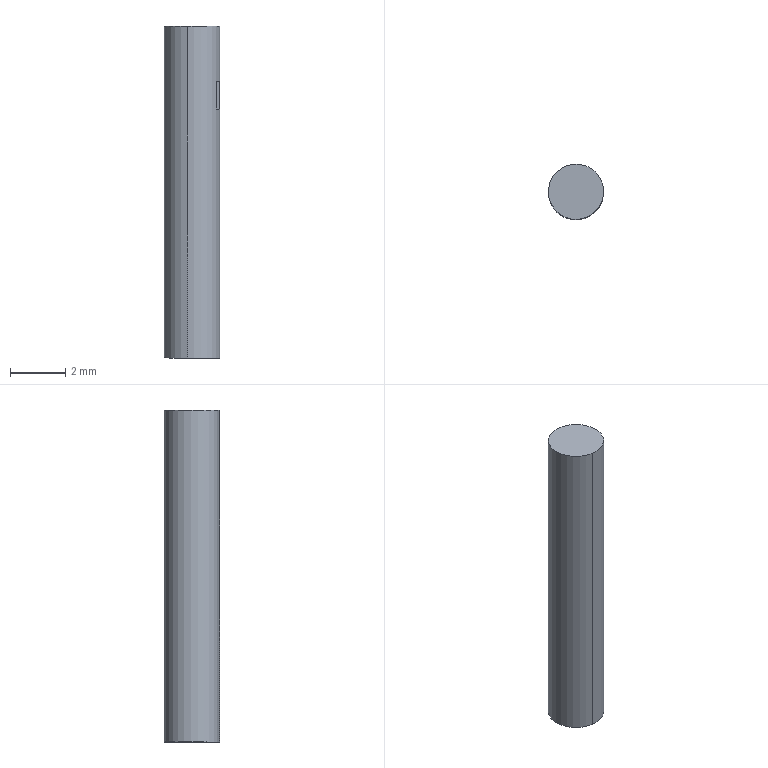Component | SolidWorks | RearAxis-1 | 1 solid | 9 faces | box 2 x 2 x 12 mm | volume 38 mm3 | plane 7 | cylinder 2 | commonest cylinder face diameters 2 x2
build123d program:
from build123d import *

# Parameters (mm, degrees)
BOSS_EXTRUDE1_DEPTH      = 5
BOSS_EXTRUDE1_DEPTH_BACK = 7
SKETCH2_R                = 1
CUT_EXTRUDE1_START       = -2
SKETCH3_W                = 0.7
SKETCH3_H                = 0.5
CUT_EXTRUDE1_DEPTH       = 1


with BuildPart() as part:
    # Sketch2 → Boss-Extrude1 (new, two sides: drawn at the far end of the back side and taken through both)
    with BuildSketch(Plane.XY.offset(-BOSS_EXTRUDE1_DEPTH_BACK)):
        with Locations((-5, 0)):
            Circle(SKETCH2_R)
    extrude(amount=BOSS_EXTRUDE1_DEPTH + BOSS_EXTRUDE1_DEPTH_BACK)

    # Sketch3 → Cut-Extrude1 (cut)
    with BuildSketch(Plane.XY.offset(5).offset(CUT_EXTRUDE1_START)):
        with Locations((-5, 1)):
            Rectangle(SKETCH3_W, SKETCH3_H)
    extrude(amount=-CUT_EXTRUDE1_DEPTH, mode=Mode.SUBTRACT)


solid = part.part

# Placed as in the assembly
solid = solid.moved(Location((11.697, -8.435, 2), (0, 0, -99.237)))
STEP:
#1=CARTESIAN_POINT('',(0.5307,-0.1301,0.1575));
#2=VERTEX_POINT('',#1);
#3=CARTESIAN_POINT('',(0.5307,-0.1301,0.1969));
#4=VERTEX_POINT('',#3);
#5=CARTESIAN_POINT('',(0.5307,-0.1301,-0.1969));
#6=DIRECTION('',(0.,-0.,1.));
#7=VECTOR('',#6,39.37);
#8=LINE('',#5,#7);
#9=EDGE_CURVE('',#2,#4,#8,.T.);
#10=ORIENTED_EDGE('',*,*,#9,.F.);
#11=CARTESIAN_POINT('',(0.5263,-0.1573,0.1575));
#12=VERTEX_POINT('',#11);
#13=CARTESIAN_POINT('',(0.4921,-0.1378,0.1575));
#14=DIRECTION('',(-0.,0.,-1.));
#15=DIRECTION('',(-0.1605,-0.987,0.));
#16=AXIS2_PLACEMENT_3D('',#13,#14,#15);
#17=CIRCLE('',#16,0.03937);
#18=EDGE_CURVE('',#2,#12,#17,.T.);
#19=ORIENTED_EDGE('',*,*,#18,.T.);
#20=CARTESIAN_POINT('',(0.5263,-0.1573,0.1969));
#21=VERTEX_POINT('',#20);
#22=CARTESIAN_POINT('',(0.5263,-0.1573,-0.1969));
#23=DIRECTION('',(-0.,0.,-1.));
#24=VECTOR('',#23,39.37);
#25=LINE('',#22,#24);
#26=EDGE_CURVE('',#21,#12,#25,.T.);
#27=ORIENTED_EDGE('',*,*,#26,.F.);
#28=CARTESIAN_POINT('',(0.4921,-0.1378,0.1969));
#29=DIRECTION('',(-0.,0.,-1.));
#30=DIRECTION('',(-0.1605,-0.987,0.));
#31=AXIS2_PLACEMENT_3D('',#28,#29,#30);
#32=CIRCLE('',#31,0.03937);
#33=EDGE_CURVE('',#4,#21,#32,.T.);
#34=ORIENTED_EDGE('',*,*,#33,.F.);
#35=EDGE_LOOP('',(#10,#19,#27,#34));
#36=FACE_BOUND('',#35,.T.);
#37=CARTESIAN_POINT('',(0.4858,-0.1767,-0.1969));
#38=VERTEX_POINT('',#37);
#39=CARTESIAN_POINT('',(0.4984,-0.09894,-0.1969));
#40=VERTEX_POINT('',#39);
#41=CARTESIAN_POINT('',(0.4921,-0.1378,-0.1969));
#42=DIRECTION('',(0.,-0.,1.));
#43=DIRECTION('',(-0.1605,-0.987,0.));
#44=AXIS2_PLACEMENT_3D('',#41,#42,#43);
#45=CIRCLE('',#44,0.03937);
#46=EDGE_CURVE('',#38,#40,#45,.T.);
#47=ORIENTED_EDGE('',*,*,#46,.T.);
#48=CARTESIAN_POINT('',(0.4984,-0.09894,0.2756));
#49=VERTEX_POINT('',#48);
#50=CARTESIAN_POINT('',(0.4984,-0.09894,-0.1969));
#51=DIRECTION('',(0.,-0.,1.));
#52=VECTOR('',#51,39.37);
#53=LINE('',#50,#52);
#54=EDGE_CURVE('',#40,#49,#53,.T.);
#55=ORIENTED_EDGE('',*,*,#54,.T.);
#56=CARTESIAN_POINT('',(0.4858,-0.1767,0.2756));
#57=VERTEX_POINT('',#56);
#58=CARTESIAN_POINT('',(0.4921,-0.1378,0.2756));
#59=DIRECTION('',(0.,-0.,1.));
#60=DIRECTION('',(-0.1605,-0.987,0.));
#61=AXIS2_PLACEMENT_3D('',#58,#59,#60);
#62=CIRCLE('',#61,0.03937);
#63=EDGE_CURVE('',#57,#49,#62,.T.);
#64=ORIENTED_EDGE('',*,*,#63,.F.);
#65=CARTESIAN_POINT('',(0.4858,-0.1767,-0.1969));
#66=DIRECTION('',(0.,-0.,1.));
#67=VECTOR('',#66,39.37);
#68=LINE('',#65,#67);
#69=EDGE_CURVE('',#38,#57,#68,.T.);
#70=ORIENTED_EDGE('',*,*,#69,.F.);
#71=EDGE_LOOP('',(#47,#55,#64,#70));
#72=FACE_OUTER_BOUND('',#71,.T.);
#73=CARTESIAN_POINT('',(0.4921,-0.1378,-0.1969));
#74=DIRECTION('',(0.,-0.,1.));
#75=DIRECTION('',(-0.1605,-0.987,0.));
#76=AXIS2_PLACEMENT_3D('',#73,#74,#75);
#77=CYLINDRICAL_SURFACE('',#76,0.03937);
#78=ADVANCED_FACE('',(#36,#72),#77,.T.);
#79=ORIENTED_EDGE('',*,*,#54,.F.);
#80=CARTESIAN_POINT('',(0.4921,-0.1378,-0.1969));
#81=DIRECTION('',(0.,-0.,1.));
#82=DIRECTION('',(-0.1605,-0.987,0.));
#83=AXIS2_PLACEMENT_3D('',#80,#81,#82);
#84=CIRCLE('',#83,0.03937);
#85=EDGE_CURVE('',#40,#38,#84,.T.);
#86=ORIENTED_EDGE('',*,*,#85,.T.);
#87=ORIENTED_EDGE('',*,*,#69,.T.);
#88=CARTESIAN_POINT('',(0.4921,-0.1378,0.2756));
#89=DIRECTION('',(0.,-0.,1.));
#90=DIRECTION('',(-0.1605,-0.987,0.));
#91=AXIS2_PLACEMENT_3D('',#88,#89,#90);
#92=CIRCLE('',#91,0.03937);
#93=EDGE_CURVE('',#49,#57,#92,.T.);
#94=ORIENTED_EDGE('',*,*,#93,.F.);
#95=EDGE_LOOP('',(#79,#86,#87,#94));
#96=FACE_OUTER_BOUND('',#95,.T.);
#97=CARTESIAN_POINT('',(0.4921,-0.1378,-0.1969));
#98=DIRECTION('',(0.,-0.,1.));
#99=DIRECTION('',(-0.1605,-0.987,0.));
#100=AXIS2_PLACEMENT_3D('',#97,#98,#99);
#101=CYLINDRICAL_SURFACE('',#100,0.03937);
#102=ADVANCED_FACE('',(#96),#101,.T.);
#103=ORIENTED_EDGE('',*,*,#46,.F.);
#104=ORIENTED_EDGE('',*,*,#85,.F.);
#105=EDGE_LOOP('',(#103,#104));
#106=FACE_OUTER_BOUND('',#105,.T.);
#107=CARTESIAN_POINT('',(0.4921,-0.1378,-0.1969));
#108=DIRECTION('',(0.,-0.,1.));
#109=DIRECTION('',(-0.1605,-0.987,-0.));
#110=AXIS2_PLACEMENT_3D('',#107,#108,#109);
#111=PLANE('',#110);
#112=ADVANCED_FACE('',(#106),#111,.F.);
#113=ORIENTED_EDGE('',*,*,#63,.T.);
#114=ORIENTED_EDGE('',*,*,#93,.T.);
#115=EDGE_LOOP('',(#113,#114));
#116=FACE_OUTER_BOUND('',#115,.T.);
#117=CARTESIAN_POINT('',(0.4921,-0.1378,0.2756));
#118=DIRECTION('',(0.,-0.,1.));
#119=DIRECTION('',(-0.1605,-0.987,-0.));
#120=AXIS2_PLACEMENT_3D('',#117,#118,#119);
#121=PLANE('',#120);
#122=ADVANCED_FACE('',(#116),#121,.T.);
#123=ORIENTED_EDGE('',*,*,#26,.T.);
#124=CARTESIAN_POINT('',(0.5191,-0.1561,0.1575));
#125=VERTEX_POINT('',#124);
#126=CARTESIAN_POINT('',(0.5385,-0.1593,0.1575));
#127=DIRECTION('',(0.987,-0.1605,-0.));
#128=VECTOR('',#127,39.37);
#129=LINE('',#126,#128);
#130=EDGE_CURVE('',#125,#12,#129,.T.);
#131=ORIENTED_EDGE('',*,*,#130,.F.);
#132=CARTESIAN_POINT('',(0.5191,-0.1561,0.1969));
#133=VERTEX_POINT('',#132);
#134=CARTESIAN_POINT('',(0.5191,-0.1561,0.1575));
#135=DIRECTION('',(0.,-0.,1.));
#136=VECTOR('',#135,39.37);
#137=LINE('',#134,#136);
#138=EDGE_CURVE('',#125,#133,#137,.T.);
#139=ORIENTED_EDGE('',*,*,#138,.T.);
#140=CARTESIAN_POINT('',(0.5385,-0.1593,0.1969));
#141=DIRECTION('',(0.987,-0.1605,-0.));
#142=VECTOR('',#141,39.37);
#143=LINE('',#140,#142);
#144=EDGE_CURVE('',#133,#21,#143,.T.);
#145=ORIENTED_EDGE('',*,*,#144,.T.);
#146=EDGE_LOOP('',(#123,#131,#139,#145));
#147=FACE_OUTER_BOUND('',#146,.T.);
#148=CARTESIAN_POINT('',(0.5385,-0.1593,0.1575));
#149=DIRECTION('',(-0.1605,-0.987,-0.));
#150=DIRECTION('',(-0.,0.,-1.));
#151=AXIS2_PLACEMENT_3D('',#148,#149,#150);
#152=PLANE('',#151);
#153=ADVANCED_FACE('',(#147),#152,.F.);
#154=CARTESIAN_POINT('',(0.5235,-0.1289,0.1969));
#155=VERTEX_POINT('',#154);
#156=CARTESIAN_POINT('',(0.5235,-0.1289,0.1969));
#157=DIRECTION('',(-0.1605,-0.987,-0.));
#158=VECTOR('',#157,39.37);
#159=LINE('',#156,#158);
#160=EDGE_CURVE('',#155,#133,#159,.T.);
#161=ORIENTED_EDGE('',*,*,#160,.T.);
#162=ORIENTED_EDGE('',*,*,#138,.F.);
#163=CARTESIAN_POINT('',(0.5235,-0.1289,0.1575));
#164=VERTEX_POINT('',#163);
#165=CARTESIAN_POINT('',(0.5235,-0.1289,0.1575));
#166=DIRECTION('',(-0.1605,-0.987,-0.));
#167=VECTOR('',#166,39.37);
#168=LINE('',#165,#167);
#169=EDGE_CURVE('',#164,#125,#168,.T.);
#170=ORIENTED_EDGE('',*,*,#169,.F.);
#171=CARTESIAN_POINT('',(0.5235,-0.1289,0.1575));
#172=DIRECTION('',(0.,-0.,1.));
#173=VECTOR('',#172,39.37);
#174=LINE('',#171,#173);
#175=EDGE_CURVE('',#164,#155,#174,.T.);
#176=ORIENTED_EDGE('',*,*,#175,.T.);
#177=EDGE_LOOP('',(#161,#162,#170,#176));
#178=FACE_OUTER_BOUND('',#177,.T.);
#179=CARTESIAN_POINT('',(0.5235,-0.1289,0.1575));
#180=DIRECTION('',(-0.987,0.1605,0.));
#181=DIRECTION('',(-0.,0.,-1.));
#182=AXIS2_PLACEMENT_3D('',#179,#180,#181);
#183=PLANE('',#182);
#184=ADVANCED_FACE('',(#178),#183,.F.);
#185=ORIENTED_EDGE('',*,*,#9,.T.);
#186=CARTESIAN_POINT('',(0.5429,-0.1321,0.1969));
#187=DIRECTION('',(-0.987,0.1605,0.));
#188=VECTOR('',#187,39.37);
#189=LINE('',#186,#188);
#190=EDGE_CURVE('',#4,#155,#189,.T.);
#191=ORIENTED_EDGE('',*,*,#190,.T.);
#192=ORIENTED_EDGE('',*,*,#175,.F.);
#193=CARTESIAN_POINT('',(0.5429,-0.1321,0.1575));
#194=DIRECTION('',(-0.987,0.1605,0.));
#195=VECTOR('',#194,39.37);
#196=LINE('',#193,#195);
#197=EDGE_CURVE('',#2,#164,#196,.T.);
#198=ORIENTED_EDGE('',*,*,#197,.F.);
#199=EDGE_LOOP('',(#185,#191,#192,#198));
#200=FACE_OUTER_BOUND('',#199,.T.);
#201=CARTESIAN_POINT('',(0.5429,-0.1321,0.1575));
#202=DIRECTION('',(0.1605,0.987,0.));
#203=DIRECTION('',(0.,-0.,1.));
#204=AXIS2_PLACEMENT_3D('',#201,#202,#203);
#205=PLANE('',#204);
#206=ADVANCED_FACE('',(#200),#205,.F.);
#207=ORIENTED_EDGE('',*,*,#197,.T.);
#208=ORIENTED_EDGE('',*,*,#169,.T.);
#209=ORIENTED_EDGE('',*,*,#130,.T.);
#210=ORIENTED_EDGE('',*,*,#18,.F.);
#211=EDGE_LOOP('',(#207,#208,#209,#210));
#212=FACE_OUTER_BOUND('',#211,.T.);
#213=CARTESIAN_POINT('',(0.4605,-0.3321,0.1575));
#214=DIRECTION('',(0.,-0.,1.));
#215=DIRECTION('',(-0.1605,-0.987,-0.));
#216=AXIS2_PLACEMENT_3D('',#213,#214,#215);
#217=PLANE('',#216);
#218=ADVANCED_FACE('',(#212),#217,.T.);
#219=ORIENTED_EDGE('',*,*,#33,.T.);
#220=ORIENTED_EDGE('',*,*,#144,.F.);
#221=ORIENTED_EDGE('',*,*,#160,.F.);
#222=ORIENTED_EDGE('',*,*,#190,.F.);
#223=EDGE_LOOP('',(#219,#220,#221,#222));
#224=FACE_OUTER_BOUND('',#223,.T.);
#225=CARTESIAN_POINT('',(0.4605,-0.3321,0.1969));
#226=DIRECTION('',(0.,-0.,1.));
#227=DIRECTION('',(-0.1605,-0.987,-0.));
#228=AXIS2_PLACEMENT_3D('',#225,#226,#227);
#229=PLANE('',#228);
#230=ADVANCED_FACE('',(#224),#229,.F.);
#231=CLOSED_SHELL('',(#78,#102,#112,#122,#153,#184,#206,#218,#230));
#232=MANIFOLD_SOLID_BREP('',#231);
#233=CARTESIAN_POINT('',(0.,0.,0.));
#234=DIRECTION('',(0.,0.,1.));
#235=DIRECTION('',(1.,0.,0.));
#236=AXIS2_PLACEMENT_3D('',#233,#234,#235);
#237=(LENGTH_UNIT()NAMED_UNIT(*)SI_UNIT($,.METRE.));
#238=LENGTH_MEASURE_WITH_UNIT(LENGTH_MEASURE(0.0254),#237);
#239=DIMENSIONAL_EXPONENTS(1.,0.,0.,0.,0.,0.,0.);
#240=(CONVERSION_BASED_UNIT('',#238)LENGTH_UNIT()NAMED_UNIT(#239));
#241=UNCERTAINTY_MEASURE_WITH_UNIT(LENGTH_MEASURE(0.00001),#240,'','');
#242=(NAMED_UNIT(*)PLANE_ANGLE_UNIT()SI_UNIT($,.RADIAN.));
#243=(NAMED_UNIT(*)SI_UNIT($,.STERADIAN.)SOLID_ANGLE_UNIT());
#244=(GEOMETRIC_REPRESENTATION_CONTEXT(3)GLOBAL_UNCERTAINTY_ASSIGNED_CONTEXT((#241))GLOBAL_UNIT_ASSIGNED_CONTEXT((#240,#242,#243))REPRESENTATION_CONTEXT('',''));
#245=ADVANCED_BREP_SHAPE_REPRESENTATION('',(#232,#236),#244);
#246=COLOUR_RGB('',0.7922,0.8196,0.9333);
#247=FILL_AREA_STYLE_COLOUR('',#246);
#248=FILL_AREA_STYLE('',(#247));
#249=SURFACE_STYLE_FILL_AREA(#248);
#250=SURFACE_SIDE_STYLE('',(#249));
#251=SURFACE_STYLE_USAGE(.BOTH.,#250);
#252=PRESENTATION_STYLE_ASSIGNMENT((#251));
#253=STYLED_ITEM('',(#252),#232);
#254=PRESENTATION_LAYER_ASSIGNMENT('','',(#253));
#255=(LENGTH_UNIT()NAMED_UNIT(*)SI_UNIT($,.METRE.));
#256=LENGTH_MEASURE_WITH_UNIT(LENGTH_MEASURE(0.0254),#255);
#257=DIMENSIONAL_EXPONENTS(1.,0.,0.,0.,0.,0.,0.);
#258=(CONVERSION_BASED_UNIT('',#256)LENGTH_UNIT()NAMED_UNIT(#257));
#259=UNCERTAINTY_MEASURE_WITH_UNIT(LENGTH_MEASURE(0.00001),#258,'','');
#260=(NAMED_UNIT(*)PLANE_ANGLE_UNIT()SI_UNIT($,.RADIAN.));
#261=(NAMED_UNIT(*)SI_UNIT($,.STERADIAN.)SOLID_ANGLE_UNIT());
#262=(GEOMETRIC_REPRESENTATION_CONTEXT(3)GLOBAL_UNCERTAINTY_ASSIGNED_CONTEXT((#259))GLOBAL_UNIT_ASSIGNED_CONTEXT((#258,#260,#261))REPRESENTATION_CONTEXT('',''));
#263=MECHANICAL_DESIGN_GEOMETRIC_PRESENTATION_REPRESENTATION('',(#253),#262);